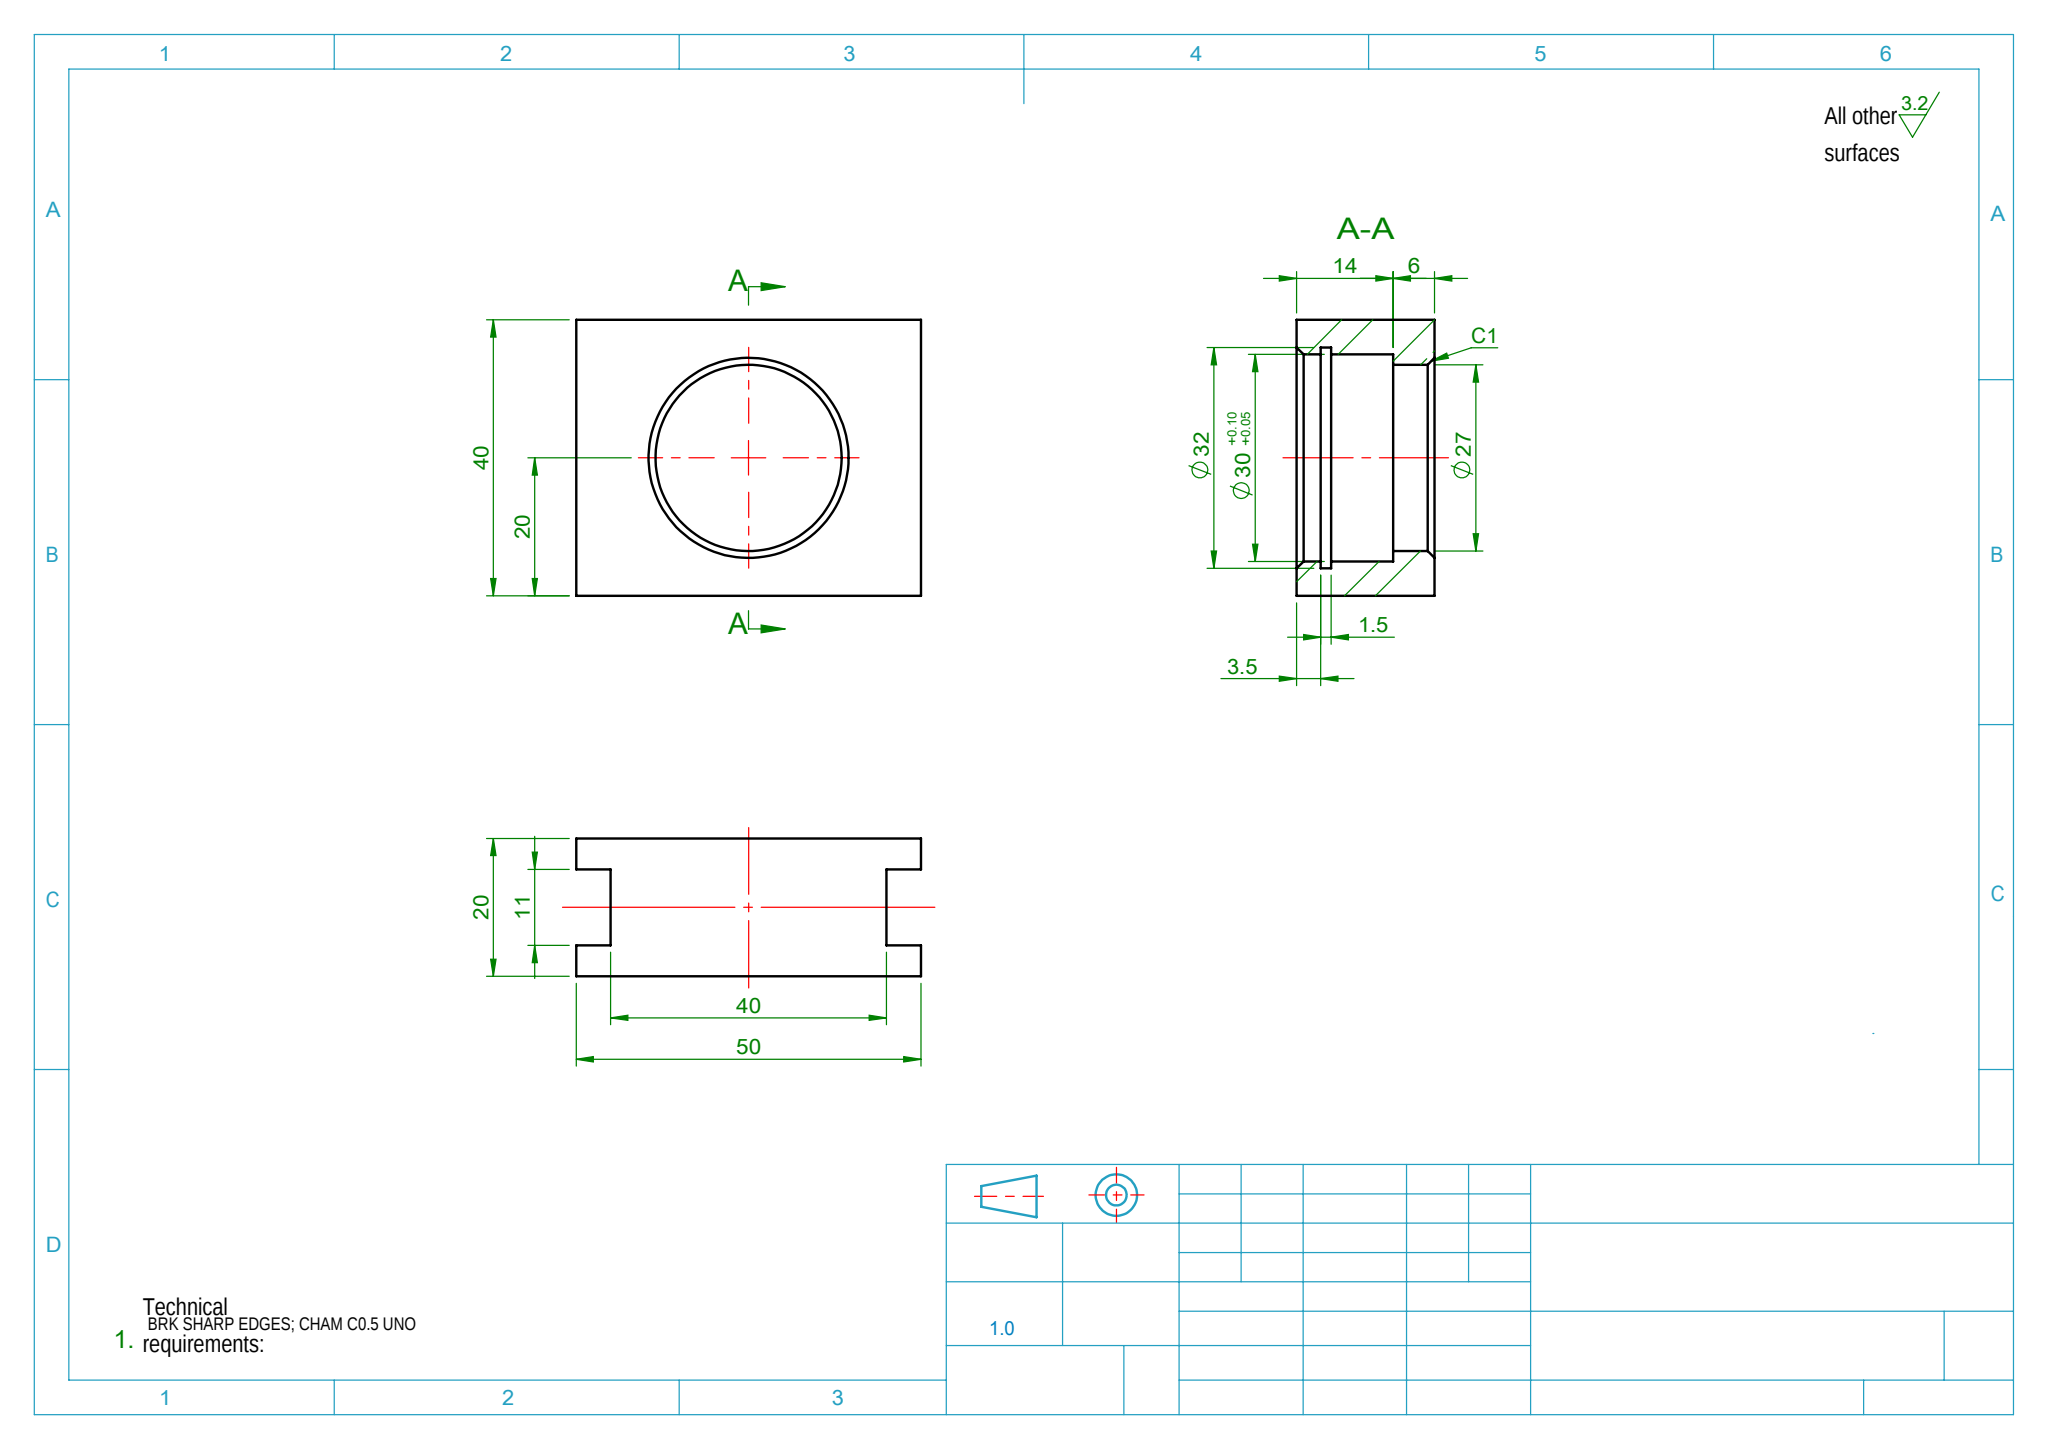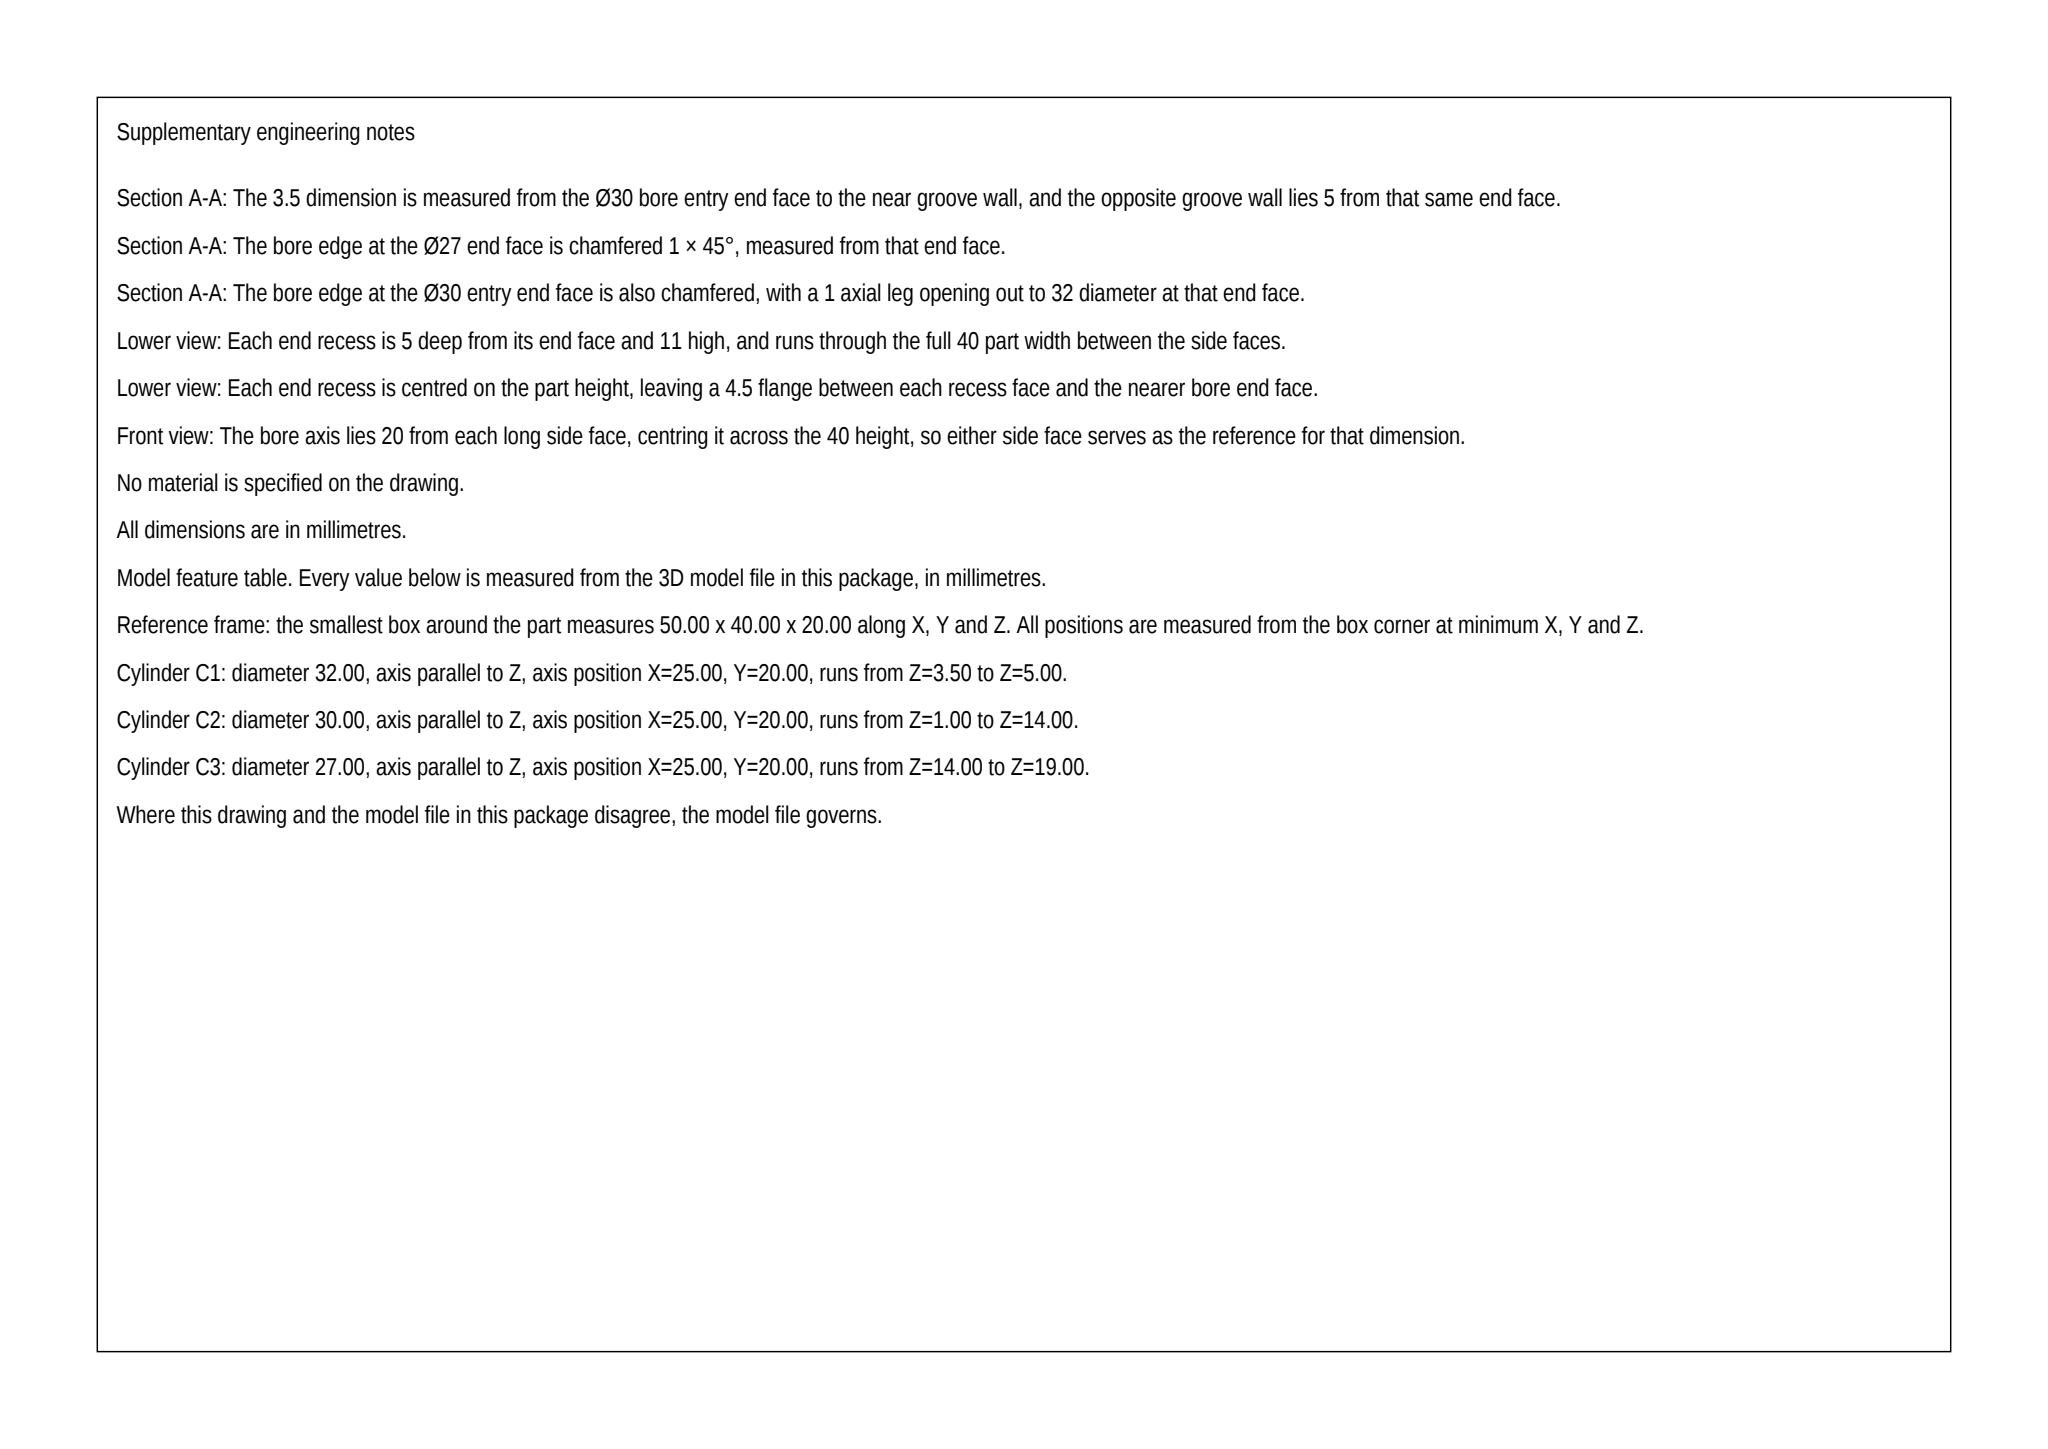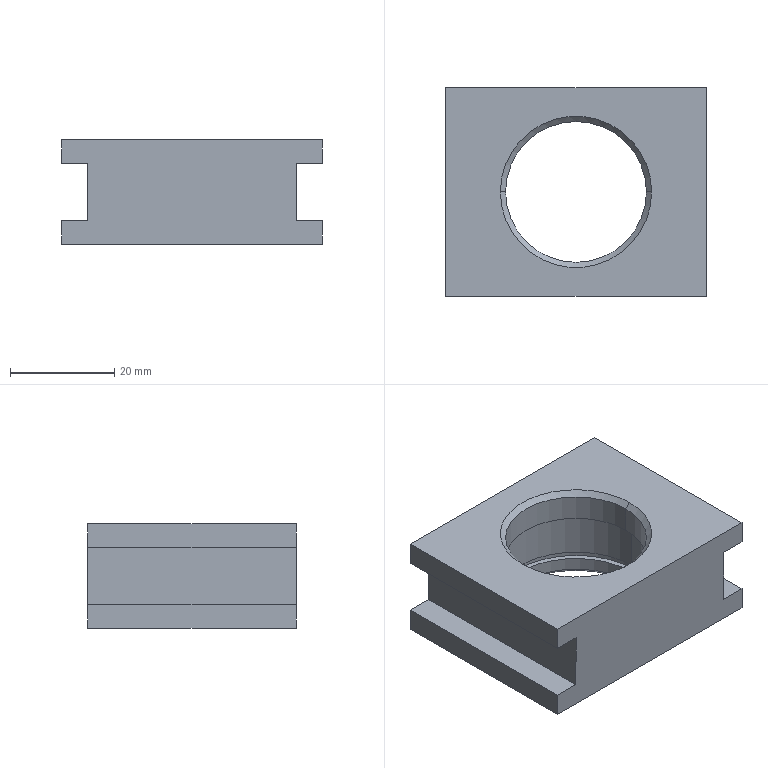Part | SolidWorks | mm | 1 solid | 29 faces | box 50 x 40 x 20 mm | volume 22031 mm3 | plane 17 | cylinder 8 | cone 4 | commonest cylinder face diameters 30 x4 32 x2 27 x2
Drawing notes:
FRONT VIEW: STEPPED BORE AXIS 25 FROM LH END FACE (CL OF 50) | from the solid: Cylinders Ø27/Ø30/Ø32 axis at x=25.0 of 50.0 bbox width
build123d program:
from build123d import *

# Parameters (mm, degrees)
SKETCH1_W           = 50
SKETCH1_H           = 40
BOSS_EXTRUDE1_DEPTH = 20
SKETCH2_W           = 5
SKETCH2_H           = 11
CUT_EXTRUDE1_DEPTH  = 52.235
SKETCH3_R           = 13.5
CUT_EXTRUDE2_DEPTH  = 38.749
SKETCH4_R           = 15
CUT_EXTRUDE3_DEPTH  = 14
SKETCH5_W           = 1
SKETCH5_H           = 1.5
CHAMFER1_SIZE       = 1


with BuildPart() as part:
    # Sketch1 → Boss-Extrude1 (new body)
    with BuildSketch(Plane.XY):
        Rectangle(SKETCH1_W, SKETCH1_H)
    extrude(amount=BOSS_EXTRUDE1_DEPTH)

    # Sketch2 → Cut-Extrude1 (cut, through all)
    with BuildSketch(Plane(origin=(0, 20, 0), x_dir=(1, 0, 0), z_dir=(0, 1, 0))):
        with Locations((-22.5, -10)):
            Rectangle(SKETCH2_W, SKETCH2_H)
        with Locations((22.5, -10)):
            Rectangle(SKETCH2_W, SKETCH2_H)
    extrude(amount=-CUT_EXTRUDE1_DEPTH, mode=Mode.SUBTRACT)

    # Sketch3 → Cut-Extrude2 (cut, through all)
    with BuildSketch(Plane.XY.offset(20)):
        Circle(SKETCH3_R)
    extrude(amount=-CUT_EXTRUDE2_DEPTH, mode=Mode.SUBTRACT)

    # Sketch4 → Cut-Extrude3 (cut)
    with BuildSketch(Plane.XY):
        Circle(SKETCH4_R)
    extrude(amount=CUT_EXTRUDE3_DEPTH, mode=Mode.SUBTRACT)

    # Sketch5 → Cut-Revolve1 (revolve, cut)
    with BuildSketch(Plane(origin=(0, 0, 0), x_dir=(1, 0, 0), z_dir=(0, 1, 0))):
        with Locations((-15.5, -4.25)):
            Rectangle(SKETCH5_W, SKETCH5_H)
    revolve(axis=Axis((0, 0, 0), (0, 0, 1)), mode=Mode.SUBTRACT)

    # Chamfer1
    chamfer1_edges = [part.edges().sort_by_distance(p)[0] for p in [
        (-13.5, 0, 20),
        (-15, 0, 0),
    ]]
    chamfer(chamfer1_edges, length=CHAMFER1_SIZE)


solid = part.part
STEP:
#1=CARTESIAN_POINT('',(15.,0.,1.));
#2=VERTEX_POINT('',#1);
#3=CARTESIAN_POINT('',(-15.,0.,1.));
#4=VERTEX_POINT('',#3);
#5=CARTESIAN_POINT('',(0.,0.,1.));
#6=DIRECTION('',(0.,0.,-1.));
#7=DIRECTION('',(1.,0.,0.));
#8=AXIS2_PLACEMENT_3D('',#5,#6,#7);
#9=CIRCLE('',#8,15.);
#10=EDGE_CURVE('',#2,#4,#9,.T.);
#11=ORIENTED_EDGE('',*,*,#10,.F.);
#12=CARTESIAN_POINT('',(16.,0.,0.));
#13=VERTEX_POINT('',#12);
#14=CARTESIAN_POINT('',(16.,0.,0.));
#15=DIRECTION('',(0.7071,0.,-0.7071));
#16=VECTOR('',#15,1000.);
#17=LINE('',#14,#16);
#18=EDGE_CURVE('',#2,#13,#17,.T.);
#19=ORIENTED_EDGE('',*,*,#18,.T.);
#20=CARTESIAN_POINT('',(-16.,0.,0.));
#21=VERTEX_POINT('',#20);
#22=CARTESIAN_POINT('',(0.,0.,0.));
#23=DIRECTION('',(0.,0.,1.));
#24=DIRECTION('',(1.,0.,0.));
#25=AXIS2_PLACEMENT_3D('',#22,#23,#24);
#26=CIRCLE('',#25,16.);
#27=EDGE_CURVE('',#21,#13,#26,.T.);
#28=ORIENTED_EDGE('',*,*,#27,.F.);
#29=CARTESIAN_POINT('',(-16.,0.,0.));
#30=DIRECTION('',(-0.7071,0.,-0.7071));
#31=VECTOR('',#30,1000.);
#32=LINE('',#29,#31);
#33=EDGE_CURVE('',#4,#21,#32,.T.);
#34=ORIENTED_EDGE('',*,*,#33,.F.);
#35=EDGE_LOOP('',(#11,#19,#28,#34));
#36=FACE_OUTER_BOUND('',#35,.T.);
#37=CARTESIAN_POINT('',(0.,0.,0.));
#38=DIRECTION('',(0.,0.,-1.));
#39=DIRECTION('',(-1.,0.,0.));
#40=AXIS2_PLACEMENT_3D('',#37,#38,#39);
#41=CONICAL_SURFACE('',#40,16.,0.7854);
#42=ADVANCED_FACE('',(#36),#41,.F.);
#43=CARTESIAN_POINT('',(-13.5,0.,19.));
#44=VERTEX_POINT('',#43);
#45=CARTESIAN_POINT('',(13.5,0.,19.));
#46=VERTEX_POINT('',#45);
#47=CARTESIAN_POINT('',(0.,0.,19.));
#48=DIRECTION('',(0.,0.,1.));
#49=DIRECTION('',(1.,0.,0.));
#50=AXIS2_PLACEMENT_3D('',#47,#48,#49);
#51=CIRCLE('',#50,13.5);
#52=EDGE_CURVE('',#44,#46,#51,.T.);
#53=ORIENTED_EDGE('',*,*,#52,.F.);
#54=CARTESIAN_POINT('',(-14.5,0.,20.));
#55=VERTEX_POINT('',#54);
#56=CARTESIAN_POINT('',(-13.5,0.,19.));
#57=DIRECTION('',(-0.7071,0.,0.7071));
#58=VECTOR('',#57,1000.);
#59=LINE('',#56,#58);
#60=EDGE_CURVE('',#44,#55,#59,.T.);
#61=ORIENTED_EDGE('',*,*,#60,.T.);
#62=CARTESIAN_POINT('',(14.5,0.,20.));
#63=VERTEX_POINT('',#62);
#64=CARTESIAN_POINT('',(0.,0.,20.));
#65=DIRECTION('',(0.,0.,-1.));
#66=DIRECTION('',(1.,0.,0.));
#67=AXIS2_PLACEMENT_3D('',#64,#65,#66);
#68=CIRCLE('',#67,14.5);
#69=EDGE_CURVE('',#63,#55,#68,.T.);
#70=ORIENTED_EDGE('',*,*,#69,.F.);
#71=CARTESIAN_POINT('',(13.5,0.,19.));
#72=DIRECTION('',(0.7071,0.,0.7071));
#73=VECTOR('',#72,1000.);
#74=LINE('',#71,#73);
#75=EDGE_CURVE('',#46,#63,#74,.T.);
#76=ORIENTED_EDGE('',*,*,#75,.F.);
#77=EDGE_LOOP('',(#53,#61,#70,#76));
#78=FACE_OUTER_BOUND('',#77,.T.);
#79=CARTESIAN_POINT('',(0.,0.,19.));
#80=DIRECTION('',(0.,0.,1.));
#81=DIRECTION('',(1.,0.,0.));
#82=AXIS2_PLACEMENT_3D('',#79,#80,#81);
#83=CONICAL_SURFACE('',#82,13.5,0.7854);
#84=ADVANCED_FACE('',(#78),#83,.F.);
#85=CARTESIAN_POINT('',(16.,0.,5.));
#86=VERTEX_POINT('',#85);
#87=CARTESIAN_POINT('',(-16.,0.,5.));
#88=VERTEX_POINT('',#87);
#89=CARTESIAN_POINT('',(0.,0.,5.));
#90=DIRECTION('',(0.,0.,-1.));
#91=DIRECTION('',(-1.,0.,0.));
#92=AXIS2_PLACEMENT_3D('',#89,#90,#91);
#93=CIRCLE('',#92,16.);
#94=EDGE_CURVE('',#86,#88,#93,.T.);
#95=ORIENTED_EDGE('',*,*,#94,.F.);
#96=CARTESIAN_POINT('',(16.,0.,3.5));
#97=VERTEX_POINT('',#96);
#98=CARTESIAN_POINT('',(16.,0.,0.));
#99=DIRECTION('',(0.,0.,-1.));
#100=VECTOR('',#99,1000.);
#101=LINE('',#98,#100);
#102=EDGE_CURVE('',#86,#97,#101,.T.);
#103=ORIENTED_EDGE('',*,*,#102,.T.);
#104=CARTESIAN_POINT('',(-16.,0.,3.5));
#105=VERTEX_POINT('',#104);
#106=CARTESIAN_POINT('',(0.,0.,3.5));
#107=DIRECTION('',(0.,0.,-1.));
#108=DIRECTION('',(-1.,0.,0.));
#109=AXIS2_PLACEMENT_3D('',#106,#107,#108);
#110=CIRCLE('',#109,16.);
#111=EDGE_CURVE('',#97,#105,#110,.T.);
#112=ORIENTED_EDGE('',*,*,#111,.T.);
#113=CARTESIAN_POINT('',(-16.,0.,0.));
#114=DIRECTION('',(0.,0.,-1.));
#115=VECTOR('',#114,1000.);
#116=LINE('',#113,#115);
#117=EDGE_CURVE('',#88,#105,#116,.T.);
#118=ORIENTED_EDGE('',*,*,#117,.F.);
#119=EDGE_LOOP('',(#95,#103,#112,#118));
#120=FACE_OUTER_BOUND('',#119,.T.);
#121=CARTESIAN_POINT('',(0.,0.,0.));
#122=DIRECTION('',(0.,0.,-1.));
#123=DIRECTION('',(-1.,0.,0.));
#124=AXIS2_PLACEMENT_3D('',#121,#122,#123);
#125=CYLINDRICAL_SURFACE('',#124,16.);
#126=ADVANCED_FACE('',(#120),#125,.F.);
#127=CARTESIAN_POINT('',(-15.,0.,14.));
#128=VERTEX_POINT('',#127);
#129=CARTESIAN_POINT('',(15.,0.,14.));
#130=VERTEX_POINT('',#129);
#131=CARTESIAN_POINT('',(0.,0.,14.));
#132=DIRECTION('',(0.,0.,1.));
#133=DIRECTION('',(1.,0.,0.));
#134=AXIS2_PLACEMENT_3D('',#131,#132,#133);
#135=CIRCLE('',#134,15.);
#136=EDGE_CURVE('',#128,#130,#135,.T.);
#137=ORIENTED_EDGE('',*,*,#136,.T.);
#138=CARTESIAN_POINT('',(15.,0.,5.));
#139=VERTEX_POINT('',#138);
#140=CARTESIAN_POINT('',(15.,0.,14.));
#141=DIRECTION('',(0.,0.,-1.));
#142=VECTOR('',#141,1000.);
#143=LINE('',#140,#142);
#144=EDGE_CURVE('',#130,#139,#143,.T.);
#145=ORIENTED_EDGE('',*,*,#144,.T.);
#146=CARTESIAN_POINT('',(-15.,0.,5.));
#147=VERTEX_POINT('',#146);
#148=CARTESIAN_POINT('',(0.,0.,5.));
#149=DIRECTION('',(0.,0.,-1.));
#150=DIRECTION('',(-1.,0.,0.));
#151=AXIS2_PLACEMENT_3D('',#148,#149,#150);
#152=CIRCLE('',#151,15.);
#153=EDGE_CURVE('',#139,#147,#152,.T.);
#154=ORIENTED_EDGE('',*,*,#153,.T.);
#155=CARTESIAN_POINT('',(-15.,0.,14.));
#156=DIRECTION('',(0.,0.,-1.));
#157=VECTOR('',#156,1000.);
#158=LINE('',#155,#157);
#159=EDGE_CURVE('',#128,#147,#158,.T.);
#160=ORIENTED_EDGE('',*,*,#159,.F.);
#161=EDGE_LOOP('',(#137,#145,#154,#160));
#162=FACE_OUTER_BOUND('',#161,.T.);
#163=CARTESIAN_POINT('',(0.,0.,14.));
#164=DIRECTION('',(0.,0.,-1.));
#165=DIRECTION('',(-1.,0.,0.));
#166=AXIS2_PLACEMENT_3D('',#163,#164,#165);
#167=CYLINDRICAL_SURFACE('',#166,15.);
#168=ADVANCED_FACE('',(#162),#167,.F.);
#169=CARTESIAN_POINT('',(13.5,0.,14.));
#170=VERTEX_POINT('',#169);
#171=CARTESIAN_POINT('',(-13.5,0.,14.));
#172=VERTEX_POINT('',#171);
#173=CARTESIAN_POINT('',(0.,0.,14.));
#174=DIRECTION('',(0.,0.,-1.));
#175=DIRECTION('',(1.,0.,0.));
#176=AXIS2_PLACEMENT_3D('',#173,#174,#175);
#177=CIRCLE('',#176,13.5);
#178=EDGE_CURVE('',#170,#172,#177,.T.);
#179=ORIENTED_EDGE('',*,*,#178,.T.);
#180=CARTESIAN_POINT('',(-13.5,0.,0.));
#181=DIRECTION('',(0.,0.,1.));
#182=VECTOR('',#181,1000.);
#183=LINE('',#180,#182);
#184=EDGE_CURVE('',#172,#44,#183,.T.);
#185=ORIENTED_EDGE('',*,*,#184,.T.);
#186=ORIENTED_EDGE('',*,*,#52,.T.);
#187=CARTESIAN_POINT('',(13.5,0.,0.));
#188=DIRECTION('',(0.,0.,1.));
#189=VECTOR('',#188,1000.);
#190=LINE('',#187,#189);
#191=EDGE_CURVE('',#170,#46,#190,.T.);
#192=ORIENTED_EDGE('',*,*,#191,.F.);
#193=EDGE_LOOP('',(#179,#185,#186,#192));
#194=FACE_OUTER_BOUND('',#193,.T.);
#195=CARTESIAN_POINT('',(0.,0.,0.));
#196=DIRECTION('',(0.,0.,1.));
#197=DIRECTION('',(1.,0.,0.));
#198=AXIS2_PLACEMENT_3D('',#195,#196,#197);
#199=CYLINDRICAL_SURFACE('',#198,13.5);
#200=ADVANCED_FACE('',(#194),#199,.F.);
#201=CARTESIAN_POINT('',(15.,0.,3.5));
#202=VERTEX_POINT('',#201);
#203=CARTESIAN_POINT('',(-15.,0.,3.5));
#204=VERTEX_POINT('',#203);
#205=CARTESIAN_POINT('',(0.,0.,3.5));
#206=DIRECTION('',(0.,0.,-1.));
#207=DIRECTION('',(-1.,0.,0.));
#208=AXIS2_PLACEMENT_3D('',#205,#206,#207);
#209=CIRCLE('',#208,15.);
#210=EDGE_CURVE('',#202,#204,#209,.T.);
#211=ORIENTED_EDGE('',*,*,#210,.F.);
#212=CARTESIAN_POINT('',(15.,0.,14.));
#213=DIRECTION('',(0.,0.,-1.));
#214=VECTOR('',#213,1000.);
#215=LINE('',#212,#214);
#216=EDGE_CURVE('',#202,#2,#215,.T.);
#217=ORIENTED_EDGE('',*,*,#216,.T.);
#218=ORIENTED_EDGE('',*,*,#10,.T.);
#219=CARTESIAN_POINT('',(-15.,0.,14.));
#220=DIRECTION('',(0.,0.,-1.));
#221=VECTOR('',#220,1000.);
#222=LINE('',#219,#221);
#223=EDGE_CURVE('',#204,#4,#222,.T.);
#224=ORIENTED_EDGE('',*,*,#223,.F.);
#225=EDGE_LOOP('',(#211,#217,#218,#224));
#226=FACE_OUTER_BOUND('',#225,.T.);
#227=CARTESIAN_POINT('',(0.,0.,14.));
#228=DIRECTION('',(0.,0.,-1.));
#229=DIRECTION('',(-1.,0.,0.));
#230=AXIS2_PLACEMENT_3D('',#227,#228,#229);
#231=CYLINDRICAL_SURFACE('',#230,15.);
#232=ADVANCED_FACE('',(#226),#231,.F.);
#233=ORIENTED_EDGE('',*,*,#216,.F.);
#234=CARTESIAN_POINT('',(0.,0.,3.5));
#235=DIRECTION('',(0.,0.,-1.));
#236=DIRECTION('',(-1.,0.,0.));
#237=AXIS2_PLACEMENT_3D('',#234,#235,#236);
#238=CIRCLE('',#237,15.);
#239=EDGE_CURVE('',#204,#202,#238,.T.);
#240=ORIENTED_EDGE('',*,*,#239,.F.);
#241=ORIENTED_EDGE('',*,*,#223,.T.);
#242=CARTESIAN_POINT('',(0.,0.,1.));
#243=DIRECTION('',(0.,0.,-1.));
#244=DIRECTION('',(1.,0.,0.));
#245=AXIS2_PLACEMENT_3D('',#242,#243,#244);
#246=CIRCLE('',#245,15.);
#247=EDGE_CURVE('',#4,#2,#246,.T.);
#248=ORIENTED_EDGE('',*,*,#247,.T.);
#249=EDGE_LOOP('',(#233,#240,#241,#248));
#250=FACE_OUTER_BOUND('',#249,.T.);
#251=CARTESIAN_POINT('',(0.,0.,14.));
#252=DIRECTION('',(0.,0.,-1.));
#253=DIRECTION('',(-1.,0.,0.));
#254=AXIS2_PLACEMENT_3D('',#251,#252,#253);
#255=CYLINDRICAL_SURFACE('',#254,15.);
#256=ADVANCED_FACE('',(#250),#255,.F.);
#257=CARTESIAN_POINT('',(25.,-20.,20.));
#258=VERTEX_POINT('',#257);
#259=CARTESIAN_POINT('',(25.,-20.,15.5));
#260=VERTEX_POINT('',#259);
#261=CARTESIAN_POINT('',(25.,-20.,20.));
#262=DIRECTION('',(0.,0.,-1.));
#263=VECTOR('',#262,1000.);
#264=LINE('',#261,#263);
#265=EDGE_CURVE('',#258,#260,#264,.T.);
#266=ORIENTED_EDGE('',*,*,#265,.T.);
#267=CARTESIAN_POINT('',(25.,20.,15.5));
#268=VERTEX_POINT('',#267);
#269=CARTESIAN_POINT('',(25.,-20.,15.5));
#270=DIRECTION('',(0.,1.,0.));
#271=VECTOR('',#270,1000.);
#272=LINE('',#269,#271);
#273=EDGE_CURVE('',#260,#268,#272,.T.);
#274=ORIENTED_EDGE('',*,*,#273,.T.);
#275=CARTESIAN_POINT('',(25.,20.,20.));
#276=VERTEX_POINT('',#275);
#277=CARTESIAN_POINT('',(25.,20.,20.));
#278=DIRECTION('',(0.,0.,-1.));
#279=VECTOR('',#278,1000.);
#280=LINE('',#277,#279);
#281=EDGE_CURVE('',#276,#268,#280,.T.);
#282=ORIENTED_EDGE('',*,*,#281,.F.);
#283=CARTESIAN_POINT('',(25.,20.,20.));
#284=DIRECTION('',(0.,1.,0.));
#285=VECTOR('',#284,1000.);
#286=LINE('',#283,#285);
#287=EDGE_CURVE('',#258,#276,#286,.T.);
#288=ORIENTED_EDGE('',*,*,#287,.F.);
#289=EDGE_LOOP('',(#266,#274,#282,#288));
#290=FACE_OUTER_BOUND('',#289,.T.);
#291=CARTESIAN_POINT('',(25.,20.,20.));
#292=DIRECTION('',(-1.,0.,0.));
#293=DIRECTION('',(0.,0.,1.));
#294=AXIS2_PLACEMENT_3D('',#291,#292,#293);
#295=PLANE('',#294);
#296=ADVANCED_FACE('',(#290),#295,.F.);
#297=CARTESIAN_POINT('',(-25.,20.,20.));
#298=VERTEX_POINT('',#297);
#299=CARTESIAN_POINT('',(-25.,20.,15.5));
#300=VERTEX_POINT('',#299);
#301=CARTESIAN_POINT('',(-25.,20.,20.));
#302=DIRECTION('',(0.,0.,-1.));
#303=VECTOR('',#302,1000.);
#304=LINE('',#301,#303);
#305=EDGE_CURVE('',#298,#300,#304,.T.);
#306=ORIENTED_EDGE('',*,*,#305,.T.);
#307=CARTESIAN_POINT('',(-25.,-20.,15.5));
#308=VERTEX_POINT('',#307);
#309=CARTESIAN_POINT('',(-25.,-20.,15.5));
#310=DIRECTION('',(0.,1.,0.));
#311=VECTOR('',#310,1000.);
#312=LINE('',#309,#311);
#313=EDGE_CURVE('',#308,#300,#312,.T.);
#314=ORIENTED_EDGE('',*,*,#313,.F.);
#315=CARTESIAN_POINT('',(-25.,-20.,20.));
#316=VERTEX_POINT('',#315);
#317=CARTESIAN_POINT('',(-25.,-20.,20.));
#318=DIRECTION('',(0.,0.,-1.));
#319=VECTOR('',#318,1000.);
#320=LINE('',#317,#319);
#321=EDGE_CURVE('',#316,#308,#320,.T.);
#322=ORIENTED_EDGE('',*,*,#321,.F.);
#323=CARTESIAN_POINT('',(-25.,20.,20.));
#324=DIRECTION('',(0.,-1.,0.));
#325=VECTOR('',#324,1000.);
#326=LINE('',#323,#325);
#327=EDGE_CURVE('',#298,#316,#326,.T.);
#328=ORIENTED_EDGE('',*,*,#327,.F.);
#329=EDGE_LOOP('',(#306,#314,#322,#328));
#330=FACE_OUTER_BOUND('',#329,.T.);
#331=CARTESIAN_POINT('',(-25.,20.,20.));
#332=DIRECTION('',(1.,0.,0.));
#333=DIRECTION('',(0.,0.,-1.));
#334=AXIS2_PLACEMENT_3D('',#331,#332,#333);
#335=PLANE('',#334);
#336=ADVANCED_FACE('',(#330),#335,.F.);
#337=CARTESIAN_POINT('',(25.,20.,4.5));
#338=VERTEX_POINT('',#337);
#339=CARTESIAN_POINT('',(25.,20.,0.));
#340=VERTEX_POINT('',#339);
#341=CARTESIAN_POINT('',(25.,20.,20.));
#342=DIRECTION('',(0.,0.,-1.));
#343=VECTOR('',#342,1000.);
#344=LINE('',#341,#343);
#345=EDGE_CURVE('',#338,#340,#344,.T.);
#346=ORIENTED_EDGE('',*,*,#345,.F.);
#347=CARTESIAN_POINT('',(25.,-20.,4.5));
#348=VERTEX_POINT('',#347);
#349=CARTESIAN_POINT('',(25.,-20.,4.5));
#350=DIRECTION('',(0.,1.,0.));
#351=VECTOR('',#350,1000.);
#352=LINE('',#349,#351);
#353=EDGE_CURVE('',#348,#338,#352,.T.);
#354=ORIENTED_EDGE('',*,*,#353,.F.);
#355=CARTESIAN_POINT('',(25.,-20.,0.));
#356=VERTEX_POINT('',#355);
#357=CARTESIAN_POINT('',(25.,-20.,20.));
#358=DIRECTION('',(0.,0.,-1.));
#359=VECTOR('',#358,1000.);
#360=LINE('',#357,#359);
#361=EDGE_CURVE('',#348,#356,#360,.T.);
#362=ORIENTED_EDGE('',*,*,#361,.T.);
#363=CARTESIAN_POINT('',(25.,20.,0.));
#364=DIRECTION('',(0.,1.,0.));
#365=VECTOR('',#364,1000.);
#366=LINE('',#363,#365);
#367=EDGE_CURVE('',#356,#340,#366,.T.);
#368=ORIENTED_EDGE('',*,*,#367,.T.);
#369=EDGE_LOOP('',(#346,#354,#362,#368));
#370=FACE_OUTER_BOUND('',#369,.T.);
#371=CARTESIAN_POINT('',(25.,20.,20.));
#372=DIRECTION('',(-1.,0.,0.));
#373=DIRECTION('',(0.,0.,1.));
#374=AXIS2_PLACEMENT_3D('',#371,#372,#373);
#375=PLANE('',#374);
#376=ADVANCED_FACE('',(#370),#375,.F.);
#377=CARTESIAN_POINT('',(-20.,20.,15.5));
#378=VERTEX_POINT('',#377);
#379=CARTESIAN_POINT('',(-20.,20.,4.5));
#380=VERTEX_POINT('',#379);
#381=CARTESIAN_POINT('',(-20.,20.,4.5));
#382=DIRECTION('',(-0.,0.,-1.));
#383=VECTOR('',#382,1000.);
#384=LINE('',#381,#383);
#385=EDGE_CURVE('',#378,#380,#384,.T.);
#386=ORIENTED_EDGE('',*,*,#385,.F.);
#387=CARTESIAN_POINT('',(-25.,20.,15.5));
#388=DIRECTION('',(1.,0.,0.));
#389=VECTOR('',#388,1000.);
#390=LINE('',#387,#389);
#391=EDGE_CURVE('',#300,#378,#390,.T.);
#392=ORIENTED_EDGE('',*,*,#391,.F.);
#393=ORIENTED_EDGE('',*,*,#305,.F.);
#394=CARTESIAN_POINT('',(-25.,20.,20.));
#395=DIRECTION('',(-1.,0.,0.));
#396=VECTOR('',#395,1000.);
#397=LINE('',#394,#396);
#398=EDGE_CURVE('',#276,#298,#397,.T.);
#399=ORIENTED_EDGE('',*,*,#398,.F.);
#400=ORIENTED_EDGE('',*,*,#281,.T.);
#401=CARTESIAN_POINT('',(20.,20.,15.5));
#402=VERTEX_POINT('',#401);
#403=CARTESIAN_POINT('',(20.,20.,15.5));
#404=DIRECTION('',(1.,0.,0.));
#405=VECTOR('',#404,1000.);
#406=LINE('',#403,#405);
#407=EDGE_CURVE('',#402,#268,#406,.T.);
#408=ORIENTED_EDGE('',*,*,#407,.F.);
#409=CARTESIAN_POINT('',(20.,20.,4.5));
#410=VERTEX_POINT('',#409);
#411=CARTESIAN_POINT('',(20.,20.,4.5));
#412=DIRECTION('',(-0.,0.,1.));
#413=VECTOR('',#412,1000.);
#414=LINE('',#411,#413);
#415=EDGE_CURVE('',#410,#402,#414,.T.);
#416=ORIENTED_EDGE('',*,*,#415,.F.);
#417=CARTESIAN_POINT('',(20.,20.,4.5));
#418=DIRECTION('',(-1.,0.,0.));
#419=VECTOR('',#418,1000.);
#420=LINE('',#417,#419);
#421=EDGE_CURVE('',#338,#410,#420,.T.);
#422=ORIENTED_EDGE('',*,*,#421,.F.);
#423=ORIENTED_EDGE('',*,*,#345,.T.);
#424=CARTESIAN_POINT('',(-25.,20.,0.));
#425=VERTEX_POINT('',#424);
#426=CARTESIAN_POINT('',(-25.,20.,0.));
#427=DIRECTION('',(-1.,0.,0.));
#428=VECTOR('',#427,1000.);
#429=LINE('',#426,#428);
#430=EDGE_CURVE('',#340,#425,#429,.T.);
#431=ORIENTED_EDGE('',*,*,#430,.T.);
#432=CARTESIAN_POINT('',(-25.,20.,4.5));
#433=VERTEX_POINT('',#432);
#434=CARTESIAN_POINT('',(-25.,20.,20.));
#435=DIRECTION('',(0.,0.,-1.));
#436=VECTOR('',#435,1000.);
#437=LINE('',#434,#436);
#438=EDGE_CURVE('',#433,#425,#437,.T.);
#439=ORIENTED_EDGE('',*,*,#438,.F.);
#440=CARTESIAN_POINT('',(-25.,20.,4.5));
#441=DIRECTION('',(-1.,0.,0.));
#442=VECTOR('',#441,1000.);
#443=LINE('',#440,#442);
#444=EDGE_CURVE('',#380,#433,#443,.T.);
#445=ORIENTED_EDGE('',*,*,#444,.F.);
#446=EDGE_LOOP('',(#386,#392,#393,#399,#400,#408,#416,#422,#423,#431,#439,#445));
#447=FACE_OUTER_BOUND('',#446,.T.);
#448=CARTESIAN_POINT('',(-25.,20.,20.));
#449=DIRECTION('',(0.,-1.,0.));
#450=DIRECTION('',(0.,0.,-1.));
#451=AXIS2_PLACEMENT_3D('',#448,#449,#450);
#452=PLANE('',#451);
#453=ADVANCED_FACE('',(#447),#452,.F.);
#454=CARTESIAN_POINT('',(-25.,-20.,4.5));
#455=VERTEX_POINT('',#454);
#456=CARTESIAN_POINT('',(-25.,-20.,0.));
#457=VERTEX_POINT('',#456);
#458=CARTESIAN_POINT('',(-25.,-20.,20.));
#459=DIRECTION('',(0.,0.,-1.));
#460=VECTOR('',#459,1000.);
#461=LINE('',#458,#460);
#462=EDGE_CURVE('',#455,#457,#461,.T.);
#463=ORIENTED_EDGE('',*,*,#462,.F.);
#464=CARTESIAN_POINT('',(-25.,-20.,4.5));
#465=DIRECTION('',(0.,1.,0.));
#466=VECTOR('',#465,1000.);
#467=LINE('',#464,#466);
#468=EDGE_CURVE('',#455,#433,#467,.T.);
#469=ORIENTED_EDGE('',*,*,#468,.T.);
#470=ORIENTED_EDGE('',*,*,#438,.T.);
#471=CARTESIAN_POINT('',(-25.,20.,0.));
#472=DIRECTION('',(0.,-1.,0.));
#473=VECTOR('',#472,1000.);
#474=LINE('',#471,#473);
#475=EDGE_CURVE('',#425,#457,#474,.T.);
#476=ORIENTED_EDGE('',*,*,#475,.T.);
#477=EDGE_LOOP('',(#463,#469,#470,#476));
#478=FACE_OUTER_BOUND('',#477,.T.);
#479=CARTESIAN_POINT('',(-25.,20.,20.));
#480=DIRECTION('',(1.,0.,0.));
#481=DIRECTION('',(0.,0.,-1.));
#482=AXIS2_PLACEMENT_3D('',#479,#480,#481);
#483=PLANE('',#482);
#484=ADVANCED_FACE('',(#478),#483,.F.);
#485=ORIENTED_EDGE('',*,*,#321,.T.);
#486=CARTESIAN_POINT('',(-20.,-20.,15.5));
#487=VERTEX_POINT('',#486);
#488=CARTESIAN_POINT('',(-25.,-20.,15.5));
#489=DIRECTION('',(1.,0.,0.));
#490=VECTOR('',#489,1000.);
#491=LINE('',#488,#490);
#492=EDGE_CURVE('',#308,#487,#491,.T.);
#493=ORIENTED_EDGE('',*,*,#492,.T.);
#494=CARTESIAN_POINT('',(-20.,-20.,4.5));
#495=VERTEX_POINT('',#494);
#496=CARTESIAN_POINT('',(-20.,-20.,4.5));
#497=DIRECTION('',(-0.,0.,-1.));
#498=VECTOR('',#497,1000.);
#499=LINE('',#496,#498);
#500=EDGE_CURVE('',#487,#495,#499,.T.);
#501=ORIENTED_EDGE('',*,*,#500,.T.);
#502=CARTESIAN_POINT('',(-25.,-20.,4.5));
#503=DIRECTION('',(-1.,0.,0.));
#504=VECTOR('',#503,1000.);
#505=LINE('',#502,#504);
#506=EDGE_CURVE('',#495,#455,#505,.T.);
#507=ORIENTED_EDGE('',*,*,#506,.T.);
#508=ORIENTED_EDGE('',*,*,#462,.T.);
#509=CARTESIAN_POINT('',(-25.,-20.,0.));
#510=DIRECTION('',(1.,0.,0.));
#511=VECTOR('',#510,1000.);
#512=LINE('',#509,#511);
#513=EDGE_CURVE('',#457,#356,#512,.T.);
#514=ORIENTED_EDGE('',*,*,#513,.T.);
#515=ORIENTED_EDGE('',*,*,#361,.F.);
#516=CARTESIAN_POINT('',(20.,-20.,4.5));
#517=VERTEX_POINT('',#516);
#518=CARTESIAN_POINT('',(20.,-20.,4.5));
#519=DIRECTION('',(-1.,0.,0.));
#520=VECTOR('',#519,1000.);
#521=LINE('',#518,#520);
#522=EDGE_CURVE('',#348,#517,#521,.T.);
#523=ORIENTED_EDGE('',*,*,#522,.T.);
#524=CARTESIAN_POINT('',(20.,-20.,15.5));
#525=VERTEX_POINT('',#524);
#526=CARTESIAN_POINT('',(20.,-20.,4.5));
#527=DIRECTION('',(-0.,0.,1.));
#528=VECTOR('',#527,1000.);
#529=LINE('',#526,#528);
#530=EDGE_CURVE('',#517,#525,#529,.T.);
#531=ORIENTED_EDGE('',*,*,#530,.T.);
#532=CARTESIAN_POINT('',(20.,-20.,15.5));
#533=DIRECTION('',(1.,0.,0.));
#534=VECTOR('',#533,1000.);
#535=LINE('',#532,#534);
#536=EDGE_CURVE('',#525,#260,#535,.T.);
#537=ORIENTED_EDGE('',*,*,#536,.T.);
#538=ORIENTED_EDGE('',*,*,#265,.F.);
#539=CARTESIAN_POINT('',(-25.,-20.,20.));
#540=DIRECTION('',(1.,0.,0.));
#541=VECTOR('',#540,1000.);
#542=LINE('',#539,#541);
#543=EDGE_CURVE('',#316,#258,#542,.T.);
#544=ORIENTED_EDGE('',*,*,#543,.F.);
#545=EDGE_LOOP('',(#485,#493,#501,#507,#508,#514,#515,#523,#531,#537,#538,#544));
#546=FACE_OUTER_BOUND('',#545,.T.);
#547=CARTESIAN_POINT('',(-25.,-20.,20.));
#548=DIRECTION('',(0.,1.,0.));
#549=DIRECTION('',(0.,0.,1.));
#550=AXIS2_PLACEMENT_3D('',#547,#548,#549);
#551=PLANE('',#550);
#552=ADVANCED_FACE('',(#546),#551,.F.);
#553=ORIENTED_EDGE('',*,*,#69,.T.);
#554=CARTESIAN_POINT('',(0.,0.,20.));
#555=DIRECTION('',(0.,0.,-1.));
#556=DIRECTION('',(1.,0.,0.));
#557=AXIS2_PLACEMENT_3D('',#554,#555,#556);
#558=CIRCLE('',#557,14.5);
#559=EDGE_CURVE('',#55,#63,#558,.T.);
#560=ORIENTED_EDGE('',*,*,#559,.T.);
#561=EDGE_LOOP('',(#553,#560));
#562=FACE_BOUND('',#561,.T.);
#563=ORIENTED_EDGE('',*,*,#287,.T.);
#564=ORIENTED_EDGE('',*,*,#398,.T.);
#565=ORIENTED_EDGE('',*,*,#327,.T.);
#566=ORIENTED_EDGE('',*,*,#543,.T.);
#567=EDGE_LOOP('',(#563,#564,#565,#566));
#568=FACE_OUTER_BOUND('',#567,.T.);
#569=CARTESIAN_POINT('',(0.,0.,20.));
#570=DIRECTION('',(0.,0.,1.));
#571=DIRECTION('',(1.,0.,0.));
#572=AXIS2_PLACEMENT_3D('',#569,#570,#571);
#573=PLANE('',#572);
#574=ADVANCED_FACE('',(#562,#568),#573,.T.);
#575=ORIENTED_EDGE('',*,*,#27,.T.);
#576=CARTESIAN_POINT('',(0.,0.,0.));
#577=DIRECTION('',(0.,0.,1.));
#578=DIRECTION('',(1.,0.,0.));
#579=AXIS2_PLACEMENT_3D('',#576,#577,#578);
#580=CIRCLE('',#579,16.);
#581=EDGE_CURVE('',#13,#21,#580,.T.);
#582=ORIENTED_EDGE('',*,*,#581,.T.);
#583=EDGE_LOOP('',(#575,#582));
#584=FACE_BOUND('',#583,.T.);
#585=ORIENTED_EDGE('',*,*,#367,.F.);
#586=ORIENTED_EDGE('',*,*,#513,.F.);
#587=ORIENTED_EDGE('',*,*,#475,.F.);
#588=ORIENTED_EDGE('',*,*,#430,.F.);
#589=EDGE_LOOP('',(#585,#586,#587,#588));
#590=FACE_OUTER_BOUND('',#589,.T.);
#591=CARTESIAN_POINT('',(0.,0.,0.));
#592=DIRECTION('',(0.,0.,1.));
#593=DIRECTION('',(1.,0.,0.));
#594=AXIS2_PLACEMENT_3D('',#591,#592,#593);
#595=PLANE('',#594);
#596=ADVANCED_FACE('',(#584,#590),#595,.F.);
#597=ORIENTED_EDGE('',*,*,#407,.T.);
#598=ORIENTED_EDGE('',*,*,#273,.F.);
#599=ORIENTED_EDGE('',*,*,#536,.F.);
#600=CARTESIAN_POINT('',(20.,-20.,15.5));
#601=DIRECTION('',(0.,1.,0.));
#602=VECTOR('',#601,1000.);
#603=LINE('',#600,#602);
#604=EDGE_CURVE('',#525,#402,#603,.T.);
#605=ORIENTED_EDGE('',*,*,#604,.T.);
#606=EDGE_LOOP('',(#597,#598,#599,#605));
#607=FACE_OUTER_BOUND('',#606,.T.);
#608=CARTESIAN_POINT('',(20.,-20.,15.5));
#609=DIRECTION('',(0.,0.,1.));
#610=DIRECTION('',(1.,0.,0.));
#611=AXIS2_PLACEMENT_3D('',#608,#609,#610);
#612=PLANE('',#611);
#613=ADVANCED_FACE('',(#607),#612,.F.);
#614=ORIENTED_EDGE('',*,*,#415,.T.);
#615=ORIENTED_EDGE('',*,*,#604,.F.);
#616=ORIENTED_EDGE('',*,*,#530,.F.);
#617=CARTESIAN_POINT('',(20.,-20.,4.5));
#618=DIRECTION('',(0.,1.,0.));
#619=VECTOR('',#618,1000.);
#620=LINE('',#617,#619);
#621=EDGE_CURVE('',#517,#410,#620,.T.);
#622=ORIENTED_EDGE('',*,*,#621,.T.);
#623=EDGE_LOOP('',(#614,#615,#616,#622));
#624=FACE_OUTER_BOUND('',#623,.T.);
#625=CARTESIAN_POINT('',(20.,-20.,4.5));
#626=DIRECTION('',(-1.,0.,-0.));
#627=DIRECTION('',(-0.,0.,1.));
#628=AXIS2_PLACEMENT_3D('',#625,#626,#627);
#629=PLANE('',#628);
#630=ADVANCED_FACE('',(#624),#629,.F.);
#631=ORIENTED_EDGE('',*,*,#421,.T.);
#632=ORIENTED_EDGE('',*,*,#621,.F.);
#633=ORIENTED_EDGE('',*,*,#522,.F.);
#634=ORIENTED_EDGE('',*,*,#353,.T.);
#635=EDGE_LOOP('',(#631,#632,#633,#634));
#636=FACE_OUTER_BOUND('',#635,.T.);
#637=CARTESIAN_POINT('',(20.,-20.,4.5));
#638=DIRECTION('',(0.,0.,-1.));
#639=DIRECTION('',(-1.,0.,0.));
#640=AXIS2_PLACEMENT_3D('',#637,#638,#639);
#641=PLANE('',#640);
#642=ADVANCED_FACE('',(#636),#641,.F.);
#643=ORIENTED_EDGE('',*,*,#385,.T.);
#644=CARTESIAN_POINT('',(-20.,-20.,4.5));
#645=DIRECTION('',(0.,1.,0.));
#646=VECTOR('',#645,1000.);
#647=LINE('',#644,#646);
#648=EDGE_CURVE('',#495,#380,#647,.T.);
#649=ORIENTED_EDGE('',*,*,#648,.F.);
#650=ORIENTED_EDGE('',*,*,#500,.F.);
#651=CARTESIAN_POINT('',(-20.,-20.,15.5));
#652=DIRECTION('',(0.,1.,0.));
#653=VECTOR('',#652,1000.);
#654=LINE('',#651,#653);
#655=EDGE_CURVE('',#487,#378,#654,.T.);
#656=ORIENTED_EDGE('',*,*,#655,.T.);
#657=EDGE_LOOP('',(#643,#649,#650,#656));
#658=FACE_OUTER_BOUND('',#657,.T.);
#659=CARTESIAN_POINT('',(-20.,-20.,4.5));
#660=DIRECTION('',(1.,0.,-0.));
#661=DIRECTION('',(-0.,0.,-1.));
#662=AXIS2_PLACEMENT_3D('',#659,#660,#661);
#663=PLANE('',#662);
#664=ADVANCED_FACE('',(#658),#663,.F.);
#665=ORIENTED_EDGE('',*,*,#391,.T.);
#666=ORIENTED_EDGE('',*,*,#655,.F.);
#667=ORIENTED_EDGE('',*,*,#492,.F.);
#668=ORIENTED_EDGE('',*,*,#313,.T.);
#669=EDGE_LOOP('',(#665,#666,#667,#668));
#670=FACE_OUTER_BOUND('',#669,.T.);
#671=CARTESIAN_POINT('',(-25.,-20.,15.5));
#672=DIRECTION('',(0.,0.,1.));
#673=DIRECTION('',(1.,0.,0.));
#674=AXIS2_PLACEMENT_3D('',#671,#672,#673);
#675=PLANE('',#674);
#676=ADVANCED_FACE('',(#670),#675,.F.);
#677=ORIENTED_EDGE('',*,*,#444,.T.);
#678=ORIENTED_EDGE('',*,*,#468,.F.);
#679=ORIENTED_EDGE('',*,*,#506,.F.);
#680=ORIENTED_EDGE('',*,*,#648,.T.);
#681=EDGE_LOOP('',(#677,#678,#679,#680));
#682=FACE_OUTER_BOUND('',#681,.T.);
#683=CARTESIAN_POINT('',(-25.,-20.,4.5));
#684=DIRECTION('',(0.,0.,-1.));
#685=DIRECTION('',(-1.,0.,0.));
#686=AXIS2_PLACEMENT_3D('',#683,#684,#685);
#687=PLANE('',#686);
#688=ADVANCED_FACE('',(#682),#687,.F.);
#689=ORIENTED_EDGE('',*,*,#184,.F.);
#690=CARTESIAN_POINT('',(0.,0.,14.));
#691=DIRECTION('',(0.,0.,-1.));
#692=DIRECTION('',(1.,0.,0.));
#693=AXIS2_PLACEMENT_3D('',#690,#691,#692);
#694=CIRCLE('',#693,13.5);
#695=EDGE_CURVE('',#172,#170,#694,.T.);
#696=ORIENTED_EDGE('',*,*,#695,.T.);
#697=ORIENTED_EDGE('',*,*,#191,.T.);
#698=CARTESIAN_POINT('',(0.,0.,19.));
#699=DIRECTION('',(0.,0.,1.));
#700=DIRECTION('',(1.,0.,0.));
#701=AXIS2_PLACEMENT_3D('',#698,#699,#700);
#702=CIRCLE('',#701,13.5);
#703=EDGE_CURVE('',#46,#44,#702,.T.);
#704=ORIENTED_EDGE('',*,*,#703,.T.);
#705=EDGE_LOOP('',(#689,#696,#697,#704));
#706=FACE_OUTER_BOUND('',#705,.T.);
#707=CARTESIAN_POINT('',(0.,0.,0.));
#708=DIRECTION('',(0.,0.,1.));
#709=DIRECTION('',(1.,0.,0.));
#710=AXIS2_PLACEMENT_3D('',#707,#708,#709);
#711=CYLINDRICAL_SURFACE('',#710,13.5);
#712=ADVANCED_FACE('',(#706),#711,.F.);
#713=ORIENTED_EDGE('',*,*,#136,.F.);
#714=CARTESIAN_POINT('',(0.,0.,14.));
#715=DIRECTION('',(0.,0.,1.));
#716=DIRECTION('',(1.,0.,0.));
#717=AXIS2_PLACEMENT_3D('',#714,#715,#716);
#718=CIRCLE('',#717,15.);
#719=EDGE_CURVE('',#130,#128,#718,.T.);
#720=ORIENTED_EDGE('',*,*,#719,.F.);
#721=EDGE_LOOP('',(#713,#720));
#722=FACE_OUTER_BOUND('',#721,.T.);
#723=ORIENTED_EDGE('',*,*,#178,.F.);
#724=ORIENTED_EDGE('',*,*,#695,.F.);
#725=EDGE_LOOP('',(#723,#724));
#726=FACE_BOUND('',#725,.T.);
#727=CARTESIAN_POINT('',(0.,0.,14.));
#728=DIRECTION('',(0.,0.,1.));
#729=DIRECTION('',(1.,0.,0.));
#730=AXIS2_PLACEMENT_3D('',#727,#728,#729);
#731=PLANE('',#730);
#732=ADVANCED_FACE('',(#722,#726),#731,.F.);
#733=ORIENTED_EDGE('',*,*,#144,.F.);
#734=ORIENTED_EDGE('',*,*,#719,.T.);
#735=ORIENTED_EDGE('',*,*,#159,.T.);
#736=CARTESIAN_POINT('',(0.,0.,5.));
#737=DIRECTION('',(0.,0.,-1.));
#738=DIRECTION('',(-1.,0.,0.));
#739=AXIS2_PLACEMENT_3D('',#736,#737,#738);
#740=CIRCLE('',#739,15.);
#741=EDGE_CURVE('',#147,#139,#740,.T.);
#742=ORIENTED_EDGE('',*,*,#741,.T.);
#743=EDGE_LOOP('',(#733,#734,#735,#742));
#744=FACE_OUTER_BOUND('',#743,.T.);
#745=CARTESIAN_POINT('',(0.,0.,14.));
#746=DIRECTION('',(0.,0.,-1.));
#747=DIRECTION('',(-1.,0.,0.));
#748=AXIS2_PLACEMENT_3D('',#745,#746,#747);
#749=CYLINDRICAL_SURFACE('',#748,15.);
#750=ADVANCED_FACE('',(#744),#749,.F.);
#751=CARTESIAN_POINT('',(0.,0.,3.5));
#752=DIRECTION('',(0.,0.,-1.));
#753=DIRECTION('',(-1.,0.,0.));
#754=AXIS2_PLACEMENT_3D('',#751,#752,#753);
#755=CIRCLE('',#754,16.);
#756=EDGE_CURVE('',#105,#97,#755,.T.);
#757=ORIENTED_EDGE('',*,*,#756,.F.);
#758=ORIENTED_EDGE('',*,*,#111,.F.);
#759=EDGE_LOOP('',(#757,#758));
#760=FACE_OUTER_BOUND('',#759,.T.);
#761=ORIENTED_EDGE('',*,*,#239,.T.);
#762=ORIENTED_EDGE('',*,*,#210,.T.);
#763=EDGE_LOOP('',(#761,#762));
#764=FACE_BOUND('',#763,.T.);
#765=CARTESIAN_POINT('',(-16.,0.,3.5));
#766=DIRECTION('',(0.,0.,-1.));
#767=DIRECTION('',(-1.,0.,0.));
#768=AXIS2_PLACEMENT_3D('',#765,#766,#767);
#769=PLANE('',#768);
#770=ADVANCED_FACE('',(#760,#764),#769,.F.);
#771=ORIENTED_EDGE('',*,*,#102,.F.);
#772=CARTESIAN_POINT('',(0.,0.,5.));
#773=DIRECTION('',(0.,0.,-1.));
#774=DIRECTION('',(-1.,0.,0.));
#775=AXIS2_PLACEMENT_3D('',#772,#773,#774);
#776=CIRCLE('',#775,16.);
#777=EDGE_CURVE('',#88,#86,#776,.T.);
#778=ORIENTED_EDGE('',*,*,#777,.F.);
#779=ORIENTED_EDGE('',*,*,#117,.T.);
#780=ORIENTED_EDGE('',*,*,#756,.T.);
#781=EDGE_LOOP('',(#771,#778,#779,#780));
#782=FACE_OUTER_BOUND('',#781,.T.);
#783=CARTESIAN_POINT('',(0.,0.,0.));
#784=DIRECTION('',(0.,0.,-1.));
#785=DIRECTION('',(-1.,0.,0.));
#786=AXIS2_PLACEMENT_3D('',#783,#784,#785);
#787=CYLINDRICAL_SURFACE('',#786,16.);
#788=ADVANCED_FACE('',(#782),#787,.F.);
#789=ORIENTED_EDGE('',*,*,#741,.F.);
#790=ORIENTED_EDGE('',*,*,#153,.F.);
#791=EDGE_LOOP('',(#789,#790));
#792=FACE_BOUND('',#791,.T.);
#793=ORIENTED_EDGE('',*,*,#777,.T.);
#794=ORIENTED_EDGE('',*,*,#94,.T.);
#795=EDGE_LOOP('',(#793,#794));
#796=FACE_OUTER_BOUND('',#795,.T.);
#797=CARTESIAN_POINT('',(-16.,0.,5.));
#798=DIRECTION('',(0.,0.,1.));
#799=DIRECTION('',(1.,0.,0.));
#800=AXIS2_PLACEMENT_3D('',#797,#798,#799);
#801=PLANE('',#800);
#802=ADVANCED_FACE('',(#792,#796),#801,.F.);
#803=ORIENTED_EDGE('',*,*,#60,.F.);
#804=ORIENTED_EDGE('',*,*,#703,.F.);
#805=ORIENTED_EDGE('',*,*,#75,.T.);
#806=ORIENTED_EDGE('',*,*,#559,.F.);
#807=EDGE_LOOP('',(#803,#804,#805,#806));
#808=FACE_OUTER_BOUND('',#807,.T.);
#809=CARTESIAN_POINT('',(0.,0.,19.));
#810=DIRECTION('',(0.,0.,1.));
#811=DIRECTION('',(1.,0.,0.));
#812=AXIS2_PLACEMENT_3D('',#809,#810,#811);
#813=CONICAL_SURFACE('',#812,13.5,0.7854);
#814=ADVANCED_FACE('',(#808),#813,.F.);
#815=ORIENTED_EDGE('',*,*,#18,.F.);
#816=ORIENTED_EDGE('',*,*,#247,.F.);
#817=ORIENTED_EDGE('',*,*,#33,.T.);
#818=ORIENTED_EDGE('',*,*,#581,.F.);
#819=EDGE_LOOP('',(#815,#816,#817,#818));
#820=FACE_OUTER_BOUND('',#819,.T.);
#821=CARTESIAN_POINT('',(0.,0.,0.));
#822=DIRECTION('',(0.,0.,-1.));
#823=DIRECTION('',(-1.,0.,0.));
#824=AXIS2_PLACEMENT_3D('',#821,#822,#823);
#825=CONICAL_SURFACE('',#824,16.,0.7854);
#826=ADVANCED_FACE('',(#820),#825,.F.);
#827=CLOSED_SHELL('',(#42,#84,#126,#168,#200,#232,#256,#296,#336,#376,#453,#484,#552,#574,#596,#613,#630,#642,#664,#676,#688,#712,#732,#750,#770,#788,#802,#814,#826));
#828=MANIFOLD_SOLID_BREP('',#827);
#829=CARTESIAN_POINT('',(0.,0.,0.));
#830=DIRECTION('',(0.,0.,1.));
#831=DIRECTION('',(1.,0.,0.));
#832=AXIS2_PLACEMENT_3D('',#829,#830,#831);
#833=(LENGTH_UNIT()NAMED_UNIT(*)SI_UNIT(.MILLI.,.METRE.));
#834=UNCERTAINTY_MEASURE_WITH_UNIT(LENGTH_MEASURE(0.00001),#833,'','');
#835=(NAMED_UNIT(*)PLANE_ANGLE_UNIT()SI_UNIT($,.RADIAN.));
#836=(NAMED_UNIT(*)SI_UNIT($,.STERADIAN.)SOLID_ANGLE_UNIT());
#837=(GEOMETRIC_REPRESENTATION_CONTEXT(3)GLOBAL_UNCERTAINTY_ASSIGNED_CONTEXT((#834))GLOBAL_UNIT_ASSIGNED_CONTEXT((#833,#835,#836))REPRESENTATION_CONTEXT('',''));
#838=ADVANCED_BREP_SHAPE_REPRESENTATION('',(#828,#832),#837);